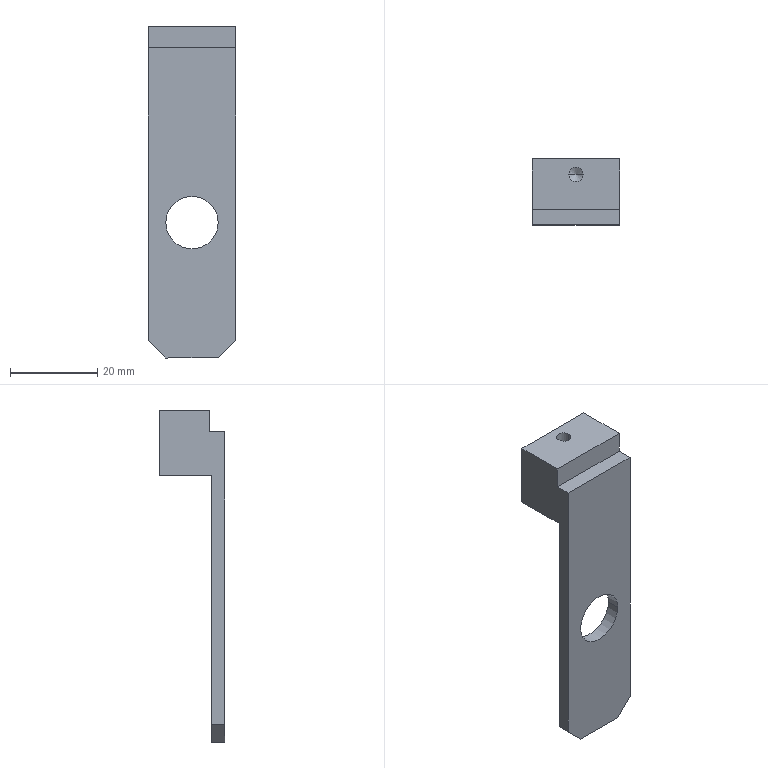Component | SolidWorks | GbgbMagnetBlockFeederF8-1 | 1 solid | 20 faces | box 20 x 15 x 76 mm | volume 7185 mm3 | plane 13 | cylinder 5 | cone 2 | commonest cylinder face diameters 12 x3 3.3 x2
build123d program:
from build123d import *

# Parameters (mm, degrees)
SKETCH1_W             = 71
SKETCH1_H             = 20
BOSS_EXTRUDE1_DEPTH   = 3
SKETCH2_W             = 10
SKETCH2_H             = 20
BOSS_EXTRUDE2_DEPTH   = 12
SKETCH3_R             = 6
CUT_EXTRUDE1_DEPTH    = 12
SKETCH6_W             = 19
SKETCH6_H             = 3
SKETCH6_H_2           = 5
BOSS_EXTRUDE3_DEPTH   = 3
SKETCH7_W             = 19
SKETCH7_H             = 5
SKETCH7_H_2           = 3
CUT_EXTRUDE2_DEPTH    = 10
SKETCH11_W            = 20
SKETCH11_H            = 15
BOSS_EXTRUDE4_DEPTH   = 5
SKETCH8_W             = 20
SKETCH8_H             = 3.5
CUT_EXTRUDE3_DEPTH    = 5
SKETCH9_R             = 6
CUT_EXTRUDE4_DEPTH    = 12
CHAMFER1_SIZE         = 4
M4_TAPPED_HOLE1_D     = 3.3
M4_TAPPED_HOLE1_DEPTH = 10.1
M4_TAPPED_HOLE1_TIP   = 0.9914


with BuildPart() as part:
    # Sketch1 → Boss-Extrude1 (new body)
    with BuildSketch(Plane(origin=(0, 0, 0), x_dir=(1, 0, 0), z_dir=(0, 1, 0))):
        Rectangle(SKETCH1_W, SKETCH1_H)
    extrude(amount=BOSS_EXTRUDE1_DEPTH)

    # Sketch2 → Boss-Extrude2 (add)
    with BuildSketch(Plane(origin=(0, 3, 0), x_dir=(1, 0, 0), z_dir=(0, 1, 0))):
        with Locations((-30.5, 0)):
            Rectangle(SKETCH2_W, SKETCH2_H)
    extrude(amount=BOSS_EXTRUDE2_DEPTH)

    # Sketch3 → Cut-Extrude1 (cut)
    with BuildSketch(Plane(origin=(0, 3, 0), x_dir=(1, 0, 0), z_dir=(0, 1, 0))):
        with Locations(Location((4.5, 0, 0), (0, 0, 270))):
            Circle(SKETCH3_R)
    extrude(amount=-CUT_EXTRUDE1_DEPTH, mode=Mode.SUBTRACT)

    # Sketch6 → Boss-Extrude3 (add)
    with BuildSketch(Plane.XZ):
        with Locations((0, 11.5)):
            Rectangle(SKETCH6_W, SKETCH6_H)
        with Locations((0, -12.5)):
            Rectangle(SKETCH6_W, SKETCH6_H_2)
    extrude(amount=-BOSS_EXTRUDE3_DEPTH)

    # Sketch7 → Cut-Extrude2 (cut)
    with BuildSketch(Plane(origin=(0, 3, 0), x_dir=(1, 0, 0), z_dir=(0, 1, 0))):
        with Locations((0, 12.5)):
            Rectangle(SKETCH7_W, SKETCH7_H)
        with Locations((0, -11.5)):
            Rectangle(SKETCH7_W, SKETCH7_H_2)
    extrude(amount=-CUT_EXTRUDE2_DEPTH, mode=Mode.SUBTRACT)

    # Sketch11 → Boss-Extrude4 (add)
    with BuildSketch(Plane.ZY.offset(35.5)):
        with Locations((0, 7.5)):
            Rectangle(SKETCH11_W, SKETCH11_H)
    extrude(amount=BOSS_EXTRUDE4_DEPTH)

    # Sketch8 → Cut-Extrude3 (cut)
    with BuildSketch(Plane.ZY.offset(40.5)):
        with Locations((0, 1.75)):
            Rectangle(SKETCH8_W, SKETCH8_H)
    extrude(amount=-CUT_EXTRUDE3_DEPTH, mode=Mode.SUBTRACT)

    # Sketch9 → Cut-Extrude4 (cut)
    with BuildSketch(Plane(origin=(0, 15, 0), x_dir=(1, 0, 0), z_dir=(0, 1, 0))):
        with Locations((-21.5, 0)):
            Circle(SKETCH9_R)
    extrude(amount=-CUT_EXTRUDE4_DEPTH, mode=Mode.SUBTRACT)

    # Chamfer1
    chamfer1_edges = [part.edges().sort_by_distance(p)[0] for p in [
        (35.5, 1.5, -10),
        (35.5, 1.5, 10),
    ]]
    chamfer(chamfer1_edges, length=CHAMFER1_SIZE)

    # M4 Tapped Hole1
    with Locations(Plane(origin=(-40.5, 4.795, -4.101), x_dir=(0, 0, 1), z_dir=(-1, 0, 0))):
        with Locations((4.101, 6.655)):
            Hole(M4_TAPPED_HOLE1_D / 2, depth=M4_TAPPED_HOLE1_DEPTH)
            with Locations((0, 0, -(M4_TAPPED_HOLE1_DEPTH + M4_TAPPED_HOLE1_TIP / 2))):  # 118° drill point
                Cone(0, M4_TAPPED_HOLE1_D / 2, M4_TAPPED_HOLE1_TIP, mode=Mode.SUBTRACT)


solid = part.part

# Placed as in the assembly
solid = solid.moved(Location((80.446, 384.34, 412.732), (0, 90, 0)))
STEP:
#1=COLOUR_RGB('',0.7922,0.8196,0.9333);
#2=FILL_AREA_STYLE_COLOUR('',#1);
#3=FILL_AREA_STYLE('',(#2));
#4=SURFACE_STYLE_FILL_AREA(#3);
#5=SURFACE_SIDE_STYLE('',(#4));
#6=SURFACE_STYLE_USAGE(.BOTH.,#5);
#7=PRESENTATION_STYLE_ASSIGNMENT((#6));
#8=CARTESIAN_POINT('',(3.102,15.582,17.446));
#9=VERTEX_POINT('',#8);
#10=CARTESIAN_POINT('',(3.232,15.582,17.446));
#11=VERTEX_POINT('',#10);
#12=CARTESIAN_POINT('',(3.167,15.582,17.446));
#13=DIRECTION('',(0.,0.,1.));
#14=DIRECTION('',(1.,0.,0.));
#15=AXIS2_PLACEMENT_3D('',#12,#13,#14);
#16=CIRCLE('',#15,0.06496);
#17=EDGE_CURVE('',#9,#11,#16,.T.);
#18=ORIENTED_EDGE('',*,*,#17,.F.);
#19=CARTESIAN_POINT('',(3.102,15.582,17.844));
#20=VERTEX_POINT('',#19);
#21=CARTESIAN_POINT('',(3.102,15.582,17.844));
#22=DIRECTION('',(0.,0.,1.));
#23=VECTOR('',#22,39.37);
#24=LINE('',#21,#23);
#25=EDGE_CURVE('',#9,#20,#24,.T.);
#26=ORIENTED_EDGE('',*,*,#25,.T.);
#27=CARTESIAN_POINT('',(3.232,15.582,17.844));
#28=VERTEX_POINT('',#27);
#29=CARTESIAN_POINT('',(3.167,15.582,17.844));
#30=DIRECTION('',(0.,0.,1.));
#31=DIRECTION('',(1.,0.,0.));
#32=AXIS2_PLACEMENT_3D('',#29,#30,#31);
#33=CIRCLE('',#32,0.06496);
#34=EDGE_CURVE('',#20,#28,#33,.T.);
#35=ORIENTED_EDGE('',*,*,#34,.T.);
#36=CARTESIAN_POINT('',(3.232,15.582,17.844));
#37=DIRECTION('',(0.,0.,1.));
#38=VECTOR('',#37,39.37);
#39=LINE('',#36,#38);
#40=EDGE_CURVE('',#11,#28,#39,.T.);
#41=ORIENTED_EDGE('',*,*,#40,.F.);
#42=EDGE_LOOP('',(#18,#26,#35,#41));
#43=FACE_OUTER_BOUND('',#42,.T.);
#44=CARTESIAN_POINT('',(3.167,15.582,17.844));
#45=DIRECTION('',(0.,0.,1.));
#46=DIRECTION('',(1.,0.,0.));
#47=AXIS2_PLACEMENT_3D('',#44,#45,#46);
#48=CYLINDRICAL_SURFACE('',#47,0.06496);
#49=ADVANCED_FACE('',(#43),#48,.F.);
#50=CARTESIAN_POINT('',(3.167,15.582,17.407));
#51=VERTEX_POINT('',#50);
#52=CARTESIAN_POINT('',(3.232,15.582,17.446));
#53=DIRECTION('',(0.8572,0.,0.515));
#54=VECTOR('',#53,39.37);
#55=LINE('',#52,#54);
#56=EDGE_CURVE('',#51,#11,#55,.T.);
#57=ORIENTED_EDGE('',*,*,#56,.F.);
#58=CARTESIAN_POINT('',(3.102,15.582,17.446));
#59=DIRECTION('',(-0.8572,-0.,0.515));
#60=VECTOR('',#59,39.37);
#61=LINE('',#58,#60);
#62=EDGE_CURVE('',#51,#9,#61,.T.);
#63=ORIENTED_EDGE('',*,*,#62,.T.);
#64=ORIENTED_EDGE('',*,*,#17,.T.);
#65=EDGE_LOOP('',(#57,#63,#64));
#66=FACE_OUTER_BOUND('',#65,.T.);
#67=CARTESIAN_POINT('',(3.167,15.582,17.446));
#68=DIRECTION('',(0.,0.,1.));
#69=DIRECTION('',(1.,0.,0.));
#70=AXIS2_PLACEMENT_3D('',#67,#68,#69);
#71=CONICAL_SURFACE('',#70,0.06496,1.03);
#72=ADVANCED_FACE('',(#66),#71,.F.);
#73=CARTESIAN_POINT('',(3.403,15.132,16.072));
#74=VERTEX_POINT('',#73);
#75=CARTESIAN_POINT('',(2.931,15.132,16.072));
#76=VERTEX_POINT('',#75);
#77=CARTESIAN_POINT('',(3.167,15.132,16.072));
#78=DIRECTION('',(0.,-1.,0.));
#79=DIRECTION('',(-1.,0.,0.));
#80=AXIS2_PLACEMENT_3D('',#77,#78,#79);
#81=CIRCLE('',#80,0.2362);
#82=EDGE_CURVE('',#74,#76,#81,.T.);
#83=ORIENTED_EDGE('',*,*,#82,.T.);
#84=CARTESIAN_POINT('',(2.931,15.25,16.072));
#85=VERTEX_POINT('',#84);
#86=CARTESIAN_POINT('',(2.931,14.777,16.072));
#87=DIRECTION('',(-0.,1.,-0.));
#88=VECTOR('',#87,39.37);
#89=LINE('',#86,#88);
#90=EDGE_CURVE('',#76,#85,#89,.T.);
#91=ORIENTED_EDGE('',*,*,#90,.T.);
#92=CARTESIAN_POINT('',(3.403,15.25,16.072));
#93=VERTEX_POINT('',#92);
#94=CARTESIAN_POINT('',(3.167,15.25,16.072));
#95=DIRECTION('',(-0.,1.,-0.));
#96=DIRECTION('',(1.,0.,0.));
#97=AXIS2_PLACEMENT_3D('',#94,#95,#96);
#98=CIRCLE('',#97,0.2362);
#99=EDGE_CURVE('',#85,#93,#98,.T.);
#100=ORIENTED_EDGE('',*,*,#99,.T.);
#101=CARTESIAN_POINT('',(3.403,14.777,16.072));
#102=DIRECTION('',(-0.,1.,-0.));
#103=VECTOR('',#102,39.37);
#104=LINE('',#101,#103);
#105=EDGE_CURVE('',#74,#93,#104,.T.);
#106=ORIENTED_EDGE('',*,*,#105,.F.);
#107=EDGE_LOOP('',(#83,#91,#100,#106));
#108=FACE_OUTER_BOUND('',#107,.T.);
#109=CARTESIAN_POINT('',(3.167,14.777,16.072));
#110=DIRECTION('',(-0.,1.,-0.));
#111=DIRECTION('',(1.,0.,0.));
#112=AXIS2_PLACEMENT_3D('',#109,#110,#111);
#113=CYLINDRICAL_SURFACE('',#112,0.2362);
#114=ADVANCED_FACE('',(#108),#113,.F.);
#115=CARTESIAN_POINT('',(3.561,15.25,17.253));
#116=VERTEX_POINT('',#115);
#117=CARTESIAN_POINT('',(3.343,15.25,17.253));
#118=VERTEX_POINT('',#117);
#119=CARTESIAN_POINT('',(2.773,15.25,17.253));
#120=DIRECTION('',(-1.,-0.,0.));
#121=VECTOR('',#120,39.37);
#122=LINE('',#119,#121);
#123=EDGE_CURVE('',#116,#118,#122,.T.);
#124=ORIENTED_EDGE('',*,*,#123,.T.);
#125=CARTESIAN_POINT('',(3.343,15.722,17.253));
#126=VERTEX_POINT('',#125);
#127=CARTESIAN_POINT('',(3.343,14.581,17.253));
#128=DIRECTION('',(-0.,1.,-0.));
#129=VECTOR('',#128,39.37);
#130=LINE('',#127,#129);
#131=EDGE_CURVE('',#118,#126,#130,.T.);
#132=ORIENTED_EDGE('',*,*,#131,.T.);
#133=CARTESIAN_POINT('',(3.561,15.722,17.253));
#134=VERTEX_POINT('',#133);
#135=CARTESIAN_POINT('',(2.773,15.722,17.253));
#136=DIRECTION('',(-1.,-0.,0.));
#137=VECTOR('',#136,39.37);
#138=LINE('',#135,#137);
#139=EDGE_CURVE('',#134,#126,#138,.T.);
#140=ORIENTED_EDGE('',*,*,#139,.F.);
#141=CARTESIAN_POINT('',(3.561,15.722,17.253));
#142=DIRECTION('',(0.,-1.,0.));
#143=VECTOR('',#142,39.37);
#144=LINE('',#141,#143);
#145=EDGE_CURVE('',#134,#116,#144,.T.);
#146=ORIENTED_EDGE('',*,*,#145,.T.);
#147=EDGE_LOOP('',(#124,#132,#140,#146));
#148=FACE_OUTER_BOUND('',#147,.T.);
#149=CARTESIAN_POINT('',(2.773,15.722,17.253));
#150=DIRECTION('',(0.,0.,1.));
#151=DIRECTION('',(1.,0.,-0.));
#152=AXIS2_PLACEMENT_3D('',#149,#150,#151);
#153=PLANE('',#152);
#154=ADVANCED_FACE('',(#148),#153,.F.);
#155=CARTESIAN_POINT('',(3.167,15.25,16.072));
#156=DIRECTION('',(-0.,1.,-0.));
#157=DIRECTION('',(1.,0.,0.));
#158=AXIS2_PLACEMENT_3D('',#155,#156,#157);
#159=CIRCLE('',#158,0.2362);
#160=EDGE_CURVE('',#93,#85,#159,.T.);
#161=ORIENTED_EDGE('',*,*,#160,.F.);
#162=ORIENTED_EDGE('',*,*,#99,.F.);
#163=EDGE_LOOP('',(#161,#162));
#164=FACE_BOUND('',#163,.T.);
#165=CARTESIAN_POINT('',(3.403,15.25,14.852));
#166=VERTEX_POINT('',#165);
#167=CARTESIAN_POINT('',(2.931,15.25,14.852));
#168=VERTEX_POINT('',#167);
#169=CARTESIAN_POINT('',(2.773,15.25,14.852));
#170=DIRECTION('',(-1.,-0.,-0.));
#171=VECTOR('',#170,39.37);
#172=LINE('',#169,#171);
#173=EDGE_CURVE('',#166,#168,#172,.T.);
#174=ORIENTED_EDGE('',*,*,#173,.T.);
#175=CARTESIAN_POINT('',(2.773,15.25,15.009));
#176=VERTEX_POINT('',#175);
#177=CARTESIAN_POINT('',(2.773,15.25,15.009));
#178=DIRECTION('',(-0.7071,-0.,0.7071));
#179=VECTOR('',#178,39.37);
#180=LINE('',#177,#179);
#181=EDGE_CURVE('',#168,#176,#180,.T.);
#182=ORIENTED_EDGE('',*,*,#181,.T.);
#183=CARTESIAN_POINT('',(2.773,15.25,17.253));
#184=VERTEX_POINT('',#183);
#185=CARTESIAN_POINT('',(2.773,15.25,14.852));
#186=DIRECTION('',(0.,0.,1.));
#187=VECTOR('',#186,39.37);
#188=LINE('',#185,#187);
#189=EDGE_CURVE('',#176,#184,#188,.T.);
#190=ORIENTED_EDGE('',*,*,#189,.T.);
#191=CARTESIAN_POINT('',(2.991,15.25,17.253));
#192=VERTEX_POINT('',#191);
#193=CARTESIAN_POINT('',(2.773,15.25,17.253));
#194=DIRECTION('',(-1.,-0.,0.));
#195=VECTOR('',#194,39.37);
#196=LINE('',#193,#195);
#197=EDGE_CURVE('',#192,#184,#196,.T.);
#198=ORIENTED_EDGE('',*,*,#197,.F.);
#199=CARTESIAN_POINT('',(3.167,15.25,17.096));
#200=DIRECTION('',(-0.,1.,-0.));
#201=DIRECTION('',(-1.,0.,0.));
#202=AXIS2_PLACEMENT_3D('',#199,#200,#201);
#203=CIRCLE('',#202,0.2362);
#204=EDGE_CURVE('',#192,#118,#203,.T.);
#205=ORIENTED_EDGE('',*,*,#204,.T.);
#206=ORIENTED_EDGE('',*,*,#123,.F.);
#207=CARTESIAN_POINT('',(3.561,15.25,15.009));
#208=VERTEX_POINT('',#207);
#209=CARTESIAN_POINT('',(3.561,15.25,14.852));
#210=DIRECTION('',(-0.,-0.,-1.));
#211=VECTOR('',#210,39.37);
#212=LINE('',#209,#211);
#213=EDGE_CURVE('',#116,#208,#212,.T.);
#214=ORIENTED_EDGE('',*,*,#213,.T.);
#215=CARTESIAN_POINT('',(3.403,15.25,14.852));
#216=DIRECTION('',(-0.7071,-0.,-0.7071));
#217=VECTOR('',#216,39.37);
#218=LINE('',#215,#217);
#219=EDGE_CURVE('',#208,#166,#218,.T.);
#220=ORIENTED_EDGE('',*,*,#219,.T.);
#221=EDGE_LOOP('',(#174,#182,#190,#198,#205,#206,#214,#220));
#222=FACE_OUTER_BOUND('',#221,.T.);
#223=CARTESIAN_POINT('',(3.167,15.25,16.249));
#224=DIRECTION('',(0.,-1.,0.));
#225=DIRECTION('',(-1.,-0.,0.));
#226=AXIS2_PLACEMENT_3D('',#223,#224,#225);
#227=PLANE('',#226);
#228=ADVANCED_FACE('',(#164,#222),#227,.F.);
#229=CARTESIAN_POINT('',(3.561,15.132,17.647));
#230=VERTEX_POINT('',#229);
#231=CARTESIAN_POINT('',(3.561,15.132,15.009));
#232=VERTEX_POINT('',#231);
#233=CARTESIAN_POINT('',(3.561,15.132,14.852));
#234=DIRECTION('',(-0.,-0.,-1.));
#235=VECTOR('',#234,39.37);
#236=LINE('',#233,#235);
#237=EDGE_CURVE('',#230,#232,#236,.T.);
#238=ORIENTED_EDGE('',*,*,#237,.T.);
#239=CARTESIAN_POINT('',(3.561,15.25,15.009));
#240=DIRECTION('',(-0.,1.,-0.));
#241=VECTOR('',#240,39.37);
#242=LINE('',#239,#241);
#243=EDGE_CURVE('',#232,#208,#242,.T.);
#244=ORIENTED_EDGE('',*,*,#243,.T.);
#245=ORIENTED_EDGE('',*,*,#213,.F.);
#246=ORIENTED_EDGE('',*,*,#145,.F.);
#247=CARTESIAN_POINT('',(3.561,15.722,17.844));
#248=VERTEX_POINT('',#247);
#249=CARTESIAN_POINT('',(3.561,15.722,17.647));
#250=DIRECTION('',(-0.,-0.,-1.));
#251=VECTOR('',#250,39.37);
#252=LINE('',#249,#251);
#253=EDGE_CURVE('',#248,#134,#252,.T.);
#254=ORIENTED_EDGE('',*,*,#253,.F.);
#255=CARTESIAN_POINT('',(3.561,15.269,17.844));
#256=VERTEX_POINT('',#255);
#257=CARTESIAN_POINT('',(3.561,15.722,17.844));
#258=DIRECTION('',(-0.,1.,-0.));
#259=VECTOR('',#258,39.37);
#260=LINE('',#257,#259);
#261=EDGE_CURVE('',#256,#248,#260,.T.);
#262=ORIENTED_EDGE('',*,*,#261,.F.);
#263=CARTESIAN_POINT('',(3.561,15.269,17.647));
#264=VERTEX_POINT('',#263);
#265=CARTESIAN_POINT('',(3.561,15.269,17.647));
#266=DIRECTION('',(0.,0.,1.));
#267=VECTOR('',#266,39.37);
#268=LINE('',#265,#267);
#269=EDGE_CURVE('',#264,#256,#268,.T.);
#270=ORIENTED_EDGE('',*,*,#269,.F.);
#271=CARTESIAN_POINT('',(3.561,15.132,17.647));
#272=DIRECTION('',(-0.,1.,-0.));
#273=VECTOR('',#272,39.37);
#274=LINE('',#271,#273);
#275=EDGE_CURVE('',#230,#264,#274,.T.);
#276=ORIENTED_EDGE('',*,*,#275,.F.);
#277=EDGE_LOOP('',(#238,#244,#245,#246,#254,#262,#270,#276));
#278=FACE_OUTER_BOUND('',#277,.T.);
#279=CARTESIAN_POINT('',(3.561,15.25,14.852));
#280=DIRECTION('',(-1.,-0.,0.));
#281=DIRECTION('',(0.,0.,1.));
#282=AXIS2_PLACEMENT_3D('',#279,#280,#281);
#283=PLANE('',#282);
#284=ADVANCED_FACE('',(#278),#283,.F.);
#285=CARTESIAN_POINT('',(3.403,15.132,14.852));
#286=VERTEX_POINT('',#285);
#287=CARTESIAN_POINT('',(2.931,15.132,14.852));
#288=VERTEX_POINT('',#287);
#289=CARTESIAN_POINT('',(2.773,15.132,14.852));
#290=DIRECTION('',(-1.,-0.,-0.));
#291=VECTOR('',#290,39.37);
#292=LINE('',#289,#291);
#293=EDGE_CURVE('',#286,#288,#292,.T.);
#294=ORIENTED_EDGE('',*,*,#293,.T.);
#295=CARTESIAN_POINT('',(2.931,15.25,14.852));
#296=DIRECTION('',(-0.,1.,-0.));
#297=VECTOR('',#296,39.37);
#298=LINE('',#295,#297);
#299=EDGE_CURVE('',#288,#168,#298,.T.);
#300=ORIENTED_EDGE('',*,*,#299,.T.);
#301=ORIENTED_EDGE('',*,*,#173,.F.);
#302=CARTESIAN_POINT('',(3.403,15.25,14.852));
#303=DIRECTION('',(0.,-1.,0.));
#304=VECTOR('',#303,39.37);
#305=LINE('',#302,#304);
#306=EDGE_CURVE('',#166,#286,#305,.T.);
#307=ORIENTED_EDGE('',*,*,#306,.T.);
#308=EDGE_LOOP('',(#294,#300,#301,#307));
#309=FACE_OUTER_BOUND('',#308,.T.);
#310=CARTESIAN_POINT('',(2.773,15.25,14.852));
#311=DIRECTION('',(-0.,-0.,1.));
#312=DIRECTION('',(1.,0.,0.));
#313=AXIS2_PLACEMENT_3D('',#310,#311,#312);
#314=PLANE('',#313);
#315=ADVANCED_FACE('',(#309),#314,.F.);
#316=ORIENTED_EDGE('',*,*,#189,.F.);
#317=CARTESIAN_POINT('',(2.773,15.132,15.009));
#318=VERTEX_POINT('',#317);
#319=CARTESIAN_POINT('',(2.773,15.25,15.009));
#320=DIRECTION('',(0.,-1.,0.));
#321=VECTOR('',#320,39.37);
#322=LINE('',#319,#321);
#323=EDGE_CURVE('',#176,#318,#322,.T.);
#324=ORIENTED_EDGE('',*,*,#323,.T.);
#325=CARTESIAN_POINT('',(2.773,15.132,17.647));
#326=VERTEX_POINT('',#325);
#327=CARTESIAN_POINT('',(2.773,15.132,14.852));
#328=DIRECTION('',(0.,0.,1.));
#329=VECTOR('',#328,39.37);
#330=LINE('',#327,#329);
#331=EDGE_CURVE('',#318,#326,#330,.T.);
#332=ORIENTED_EDGE('',*,*,#331,.T.);
#333=CARTESIAN_POINT('',(2.773,15.269,17.647));
#334=VERTEX_POINT('',#333);
#335=CARTESIAN_POINT('',(2.773,15.132,17.647));
#336=DIRECTION('',(0.,-1.,0.));
#337=VECTOR('',#336,39.37);
#338=LINE('',#335,#337);
#339=EDGE_CURVE('',#334,#326,#338,.T.);
#340=ORIENTED_EDGE('',*,*,#339,.F.);
#341=CARTESIAN_POINT('',(2.773,15.269,17.844));
#342=VERTEX_POINT('',#341);
#343=CARTESIAN_POINT('',(2.773,15.269,17.647));
#344=DIRECTION('',(0.,0.,1.));
#345=VECTOR('',#344,39.37);
#346=LINE('',#343,#345);
#347=EDGE_CURVE('',#334,#342,#346,.T.);
#348=ORIENTED_EDGE('',*,*,#347,.T.);
#349=CARTESIAN_POINT('',(2.773,15.722,17.844));
#350=VERTEX_POINT('',#349);
#351=CARTESIAN_POINT('',(2.773,15.722,17.844));
#352=DIRECTION('',(0.,-1.,0.));
#353=VECTOR('',#352,39.37);
#354=LINE('',#351,#353);
#355=EDGE_CURVE('',#350,#342,#354,.T.);
#356=ORIENTED_EDGE('',*,*,#355,.F.);
#357=CARTESIAN_POINT('',(2.773,15.722,17.253));
#358=VERTEX_POINT('',#357);
#359=CARTESIAN_POINT('',(2.773,15.722,17.647));
#360=DIRECTION('',(0.,0.,1.));
#361=VECTOR('',#360,39.37);
#362=LINE('',#359,#361);
#363=EDGE_CURVE('',#358,#350,#362,.T.);
#364=ORIENTED_EDGE('',*,*,#363,.F.);
#365=CARTESIAN_POINT('',(2.773,15.722,17.253));
#366=DIRECTION('',(0.,-1.,0.));
#367=VECTOR('',#366,39.37);
#368=LINE('',#365,#367);
#369=EDGE_CURVE('',#358,#184,#368,.T.);
#370=ORIENTED_EDGE('',*,*,#369,.T.);
#371=EDGE_LOOP('',(#316,#324,#332,#340,#348,#356,#364,#370));
#372=FACE_OUTER_BOUND('',#371,.T.);
#373=CARTESIAN_POINT('',(2.773,15.25,14.852));
#374=DIRECTION('',(1.,0.,-0.));
#375=DIRECTION('',(-0.,-0.,-1.));
#376=AXIS2_PLACEMENT_3D('',#373,#374,#375);
#377=PLANE('',#376);
#378=ADVANCED_FACE('',(#372),#377,.F.);
#379=ORIENTED_EDGE('',*,*,#331,.F.);
#380=CARTESIAN_POINT('',(2.35,15.132,15.432));
#381=DIRECTION('',(0.7071,0.,-0.7071));
#382=VECTOR('',#381,39.37);
#383=LINE('',#380,#382);
#384=EDGE_CURVE('',#318,#288,#383,.T.);
#385=ORIENTED_EDGE('',*,*,#384,.T.);
#386=ORIENTED_EDGE('',*,*,#293,.F.);
#387=CARTESIAN_POINT('',(3.984,15.132,15.432));
#388=DIRECTION('',(0.7071,0.,0.7071));
#389=VECTOR('',#388,39.37);
#390=LINE('',#387,#389);
#391=EDGE_CURVE('',#286,#232,#390,.T.);
#392=ORIENTED_EDGE('',*,*,#391,.T.);
#393=ORIENTED_EDGE('',*,*,#237,.F.);
#394=CARTESIAN_POINT('',(2.773,15.132,17.647));
#395=DIRECTION('',(1.,0.,-0.));
#396=VECTOR('',#395,39.37);
#397=LINE('',#394,#396);
#398=EDGE_CURVE('',#326,#230,#397,.T.);
#399=ORIENTED_EDGE('',*,*,#398,.F.);
#400=EDGE_LOOP('',(#379,#385,#386,#392,#393,#399));
#401=FACE_OUTER_BOUND('',#400,.T.);
#402=ORIENTED_EDGE('',*,*,#82,.F.);
#403=CARTESIAN_POINT('',(3.167,15.132,16.072));
#404=DIRECTION('',(0.,-1.,0.));
#405=DIRECTION('',(-1.,0.,0.));
#406=AXIS2_PLACEMENT_3D('',#403,#404,#405);
#407=CIRCLE('',#406,0.2362);
#408=EDGE_CURVE('',#76,#74,#407,.T.);
#409=ORIENTED_EDGE('',*,*,#408,.F.);
#410=EDGE_LOOP('',(#402,#409));
#411=FACE_BOUND('',#410,.T.);
#412=CARTESIAN_POINT('',(3.167,15.132,16.249));
#413=DIRECTION('',(0.,-1.,0.));
#414=DIRECTION('',(-1.,-0.,0.));
#415=AXIS2_PLACEMENT_3D('',#412,#413,#414);
#416=PLANE('',#415);
#417=ADVANCED_FACE('',(#401,#411),#416,.T.);
#418=CARTESIAN_POINT('',(2.991,15.722,17.253));
#419=VERTEX_POINT('',#418);
#420=CARTESIAN_POINT('',(2.773,15.722,17.253));
#421=DIRECTION('',(-1.,-0.,0.));
#422=VECTOR('',#421,39.37);
#423=LINE('',#420,#422);
#424=EDGE_CURVE('',#419,#358,#423,.T.);
#425=ORIENTED_EDGE('',*,*,#424,.F.);
#426=CARTESIAN_POINT('',(2.991,14.581,17.253));
#427=DIRECTION('',(0.,-1.,0.));
#428=VECTOR('',#427,39.37);
#429=LINE('',#426,#428);
#430=EDGE_CURVE('',#419,#192,#429,.T.);
#431=ORIENTED_EDGE('',*,*,#430,.T.);
#432=ORIENTED_EDGE('',*,*,#197,.T.);
#433=ORIENTED_EDGE('',*,*,#369,.F.);
#434=EDGE_LOOP('',(#425,#431,#432,#433));
#435=FACE_OUTER_BOUND('',#434,.T.);
#436=CARTESIAN_POINT('',(2.773,15.722,17.253));
#437=DIRECTION('',(0.,0.,1.));
#438=DIRECTION('',(1.,0.,-0.));
#439=AXIS2_PLACEMENT_3D('',#436,#437,#438);
#440=PLANE('',#439);
#441=ADVANCED_FACE('',(#435),#440,.F.);
#442=CARTESIAN_POINT('',(3.167,15.722,17.096));
#443=DIRECTION('',(-0.,1.,-0.));
#444=DIRECTION('',(1.,0.,0.));
#445=AXIS2_PLACEMENT_3D('',#442,#443,#444);
#446=CIRCLE('',#445,0.2362);
#447=EDGE_CURVE('',#419,#126,#446,.T.);
#448=ORIENTED_EDGE('',*,*,#447,.F.);
#449=ORIENTED_EDGE('',*,*,#424,.T.);
#450=ORIENTED_EDGE('',*,*,#363,.T.);
#451=CARTESIAN_POINT('',(2.773,15.722,17.844));
#452=DIRECTION('',(-1.,-0.,0.));
#453=VECTOR('',#452,39.37);
#454=LINE('',#451,#453);
#455=EDGE_CURVE('',#248,#350,#454,.T.);
#456=ORIENTED_EDGE('',*,*,#455,.F.);
#457=ORIENTED_EDGE('',*,*,#253,.T.);
#458=ORIENTED_EDGE('',*,*,#139,.T.);
#459=EDGE_LOOP('',(#448,#449,#450,#456,#457,#458));
#460=FACE_OUTER_BOUND('',#459,.T.);
#461=CARTESIAN_POINT('',(3.167,15.722,16.249));
#462=DIRECTION('',(-0.,1.,-0.));
#463=DIRECTION('',(1.,0.,-0.));
#464=AXIS2_PLACEMENT_3D('',#461,#462,#463);
#465=PLANE('',#464);
#466=ADVANCED_FACE('',(#460),#465,.T.);
#467=ORIENTED_EDGE('',*,*,#90,.F.);
#468=ORIENTED_EDGE('',*,*,#408,.T.);
#469=ORIENTED_EDGE('',*,*,#105,.T.);
#470=ORIENTED_EDGE('',*,*,#160,.T.);
#471=EDGE_LOOP('',(#467,#468,#469,#470));
#472=FACE_OUTER_BOUND('',#471,.T.);
#473=CARTESIAN_POINT('',(3.167,14.777,16.072));
#474=DIRECTION('',(-0.,1.,-0.));
#475=DIRECTION('',(1.,0.,0.));
#476=AXIS2_PLACEMENT_3D('',#473,#474,#475);
#477=CYLINDRICAL_SURFACE('',#476,0.2362);
#478=ADVANCED_FACE('',(#472),#477,.F.);
#479=CARTESIAN_POINT('',(3.167,15.582,17.844));
#480=DIRECTION('',(0.,0.,1.));
#481=DIRECTION('',(1.,0.,0.));
#482=AXIS2_PLACEMENT_3D('',#479,#480,#481);
#483=CIRCLE('',#482,0.06496);
#484=EDGE_CURVE('',#28,#20,#483,.T.);
#485=ORIENTED_EDGE('',*,*,#484,.F.);
#486=ORIENTED_EDGE('',*,*,#34,.F.);
#487=EDGE_LOOP('',(#485,#486));
#488=FACE_BOUND('',#487,.T.);
#489=CARTESIAN_POINT('',(2.773,15.269,17.844));
#490=DIRECTION('',(-1.,-0.,0.));
#491=VECTOR('',#490,39.37);
#492=LINE('',#489,#491);
#493=EDGE_CURVE('',#256,#342,#492,.T.);
#494=ORIENTED_EDGE('',*,*,#493,.F.);
#495=ORIENTED_EDGE('',*,*,#261,.T.);
#496=ORIENTED_EDGE('',*,*,#455,.T.);
#497=ORIENTED_EDGE('',*,*,#355,.T.);
#498=EDGE_LOOP('',(#494,#495,#496,#497));
#499=FACE_OUTER_BOUND('',#498,.T.);
#500=CARTESIAN_POINT('',(3.167,15.132,17.844));
#501=DIRECTION('',(0.,0.,1.));
#502=DIRECTION('',(1.,0.,-0.));
#503=AXIS2_PLACEMENT_3D('',#500,#501,#502);
#504=PLANE('',#503);
#505=ADVANCED_FACE('',(#488,#499),#504,.T.);
#506=ORIENTED_EDGE('',*,*,#493,.T.);
#507=ORIENTED_EDGE('',*,*,#347,.F.);
#508=CARTESIAN_POINT('',(2.773,15.269,17.647));
#509=DIRECTION('',(-1.,-0.,0.));
#510=VECTOR('',#509,39.37);
#511=LINE('',#508,#510);
#512=EDGE_CURVE('',#264,#334,#511,.T.);
#513=ORIENTED_EDGE('',*,*,#512,.F.);
#514=ORIENTED_EDGE('',*,*,#269,.T.);
#515=EDGE_LOOP('',(#506,#507,#513,#514));
#516=FACE_OUTER_BOUND('',#515,.T.);
#517=CARTESIAN_POINT('',(2.773,15.269,17.647));
#518=DIRECTION('',(-0.,1.,-0.));
#519=DIRECTION('',(1.,0.,-0.));
#520=AXIS2_PLACEMENT_3D('',#517,#518,#519);
#521=PLANE('',#520);
#522=ADVANCED_FACE('',(#516),#521,.F.);
#523=ORIENTED_EDGE('',*,*,#339,.T.);
#524=ORIENTED_EDGE('',*,*,#398,.T.);
#525=ORIENTED_EDGE('',*,*,#275,.T.);
#526=ORIENTED_EDGE('',*,*,#512,.T.);
#527=EDGE_LOOP('',(#523,#524,#525,#526));
#528=FACE_OUTER_BOUND('',#527,.T.);
#529=CARTESIAN_POINT('',(3.167,15.132,17.647));
#530=DIRECTION('',(-0.,-0.,-1.));
#531=DIRECTION('',(-1.,-0.,0.));
#532=AXIS2_PLACEMENT_3D('',#529,#530,#531);
#533=PLANE('',#532);
#534=ADVANCED_FACE('',(#528),#533,.F.);
#535=ORIENTED_EDGE('',*,*,#204,.F.);
#536=ORIENTED_EDGE('',*,*,#430,.F.);
#537=ORIENTED_EDGE('',*,*,#447,.T.);
#538=ORIENTED_EDGE('',*,*,#131,.F.);
#539=EDGE_LOOP('',(#535,#536,#537,#538));
#540=FACE_OUTER_BOUND('',#539,.T.);
#541=CARTESIAN_POINT('',(3.167,14.581,17.096));
#542=DIRECTION('',(-0.,1.,-0.));
#543=DIRECTION('',(1.,0.,0.));
#544=AXIS2_PLACEMENT_3D('',#541,#542,#543);
#545=CYLINDRICAL_SURFACE('',#544,0.2362);
#546=ADVANCED_FACE('',(#540),#545,.F.);
#547=ORIENTED_EDGE('',*,*,#181,.F.);
#548=ORIENTED_EDGE('',*,*,#299,.F.);
#549=ORIENTED_EDGE('',*,*,#384,.F.);
#550=ORIENTED_EDGE('',*,*,#323,.F.);
#551=EDGE_LOOP('',(#547,#548,#549,#550));
#552=FACE_OUTER_BOUND('',#551,.T.);
#553=CARTESIAN_POINT('',(2.773,15.25,15.009));
#554=DIRECTION('',(0.7071,0.,0.7071));
#555=DIRECTION('',(0.,-1.,0.));
#556=AXIS2_PLACEMENT_3D('',#553,#554,#555);
#557=PLANE('',#556);
#558=ADVANCED_FACE('',(#552),#557,.F.);
#559=ORIENTED_EDGE('',*,*,#219,.F.);
#560=ORIENTED_EDGE('',*,*,#243,.F.);
#561=ORIENTED_EDGE('',*,*,#391,.F.);
#562=ORIENTED_EDGE('',*,*,#306,.F.);
#563=EDGE_LOOP('',(#559,#560,#561,#562));
#564=FACE_OUTER_BOUND('',#563,.T.);
#565=CARTESIAN_POINT('',(3.403,15.25,14.852));
#566=DIRECTION('',(-0.7071,-0.,0.7071));
#567=DIRECTION('',(0.,-1.,0.));
#568=AXIS2_PLACEMENT_3D('',#565,#566,#567);
#569=PLANE('',#568);
#570=ADVANCED_FACE('',(#564),#569,.F.);
#571=ORIENTED_EDGE('',*,*,#62,.F.);
#572=ORIENTED_EDGE('',*,*,#56,.T.);
#573=CARTESIAN_POINT('',(3.167,15.582,17.446));
#574=DIRECTION('',(0.,0.,1.));
#575=DIRECTION('',(1.,0.,0.));
#576=AXIS2_PLACEMENT_3D('',#573,#574,#575);
#577=CIRCLE('',#576,0.06496);
#578=EDGE_CURVE('',#11,#9,#577,.T.);
#579=ORIENTED_EDGE('',*,*,#578,.T.);
#580=EDGE_LOOP('',(#571,#572,#579));
#581=FACE_OUTER_BOUND('',#580,.T.);
#582=CARTESIAN_POINT('',(3.167,15.582,17.446));
#583=DIRECTION('',(0.,0.,1.));
#584=DIRECTION('',(1.,0.,0.));
#585=AXIS2_PLACEMENT_3D('',#582,#583,#584);
#586=CONICAL_SURFACE('',#585,0.06496,1.03);
#587=ADVANCED_FACE('',(#581),#586,.F.);
#588=ORIENTED_EDGE('',*,*,#25,.F.);
#589=ORIENTED_EDGE('',*,*,#578,.F.);
#590=ORIENTED_EDGE('',*,*,#40,.T.);
#591=ORIENTED_EDGE('',*,*,#484,.T.);
#592=EDGE_LOOP('',(#588,#589,#590,#591));
#593=FACE_OUTER_BOUND('',#592,.T.);
#594=CARTESIAN_POINT('',(3.167,15.582,17.844));
#595=DIRECTION('',(0.,0.,1.));
#596=DIRECTION('',(1.,0.,0.));
#597=AXIS2_PLACEMENT_3D('',#594,#595,#596);
#598=CYLINDRICAL_SURFACE('',#597,0.06496);
#599=ADVANCED_FACE('',(#593),#598,.F.);
#600=CLOSED_SHELL('',(#49,#72,#114,#154,#228,#284,#315,#378,#417,#441,#466,#478,#505,#522,#534,#546,#558,#570,#587,#599));
#601=MANIFOLD_SOLID_BREP('',#600);
#602=STYLED_ITEM('',(#7),#601);
#603=PRESENTATION_LAYER_ASSIGNMENT('','',(#602));
#604=CARTESIAN_POINT('',(0.,0.,0.));
#605=DIRECTION('',(0.,0.,1.));
#606=DIRECTION('',(1.,0.,0.));
#607=AXIS2_PLACEMENT_3D('',#604,#605,#606);
#608=(LENGTH_UNIT()NAMED_UNIT(*)SI_UNIT($,.METRE.));
#609=LENGTH_MEASURE_WITH_UNIT(LENGTH_MEASURE(0.0254),#608);
#610=DIMENSIONAL_EXPONENTS(1.,0.,0.,0.,0.,0.,0.);
#611=(CONVERSION_BASED_UNIT('',#609)LENGTH_UNIT()NAMED_UNIT(#610));
#612=UNCERTAINTY_MEASURE_WITH_UNIT(LENGTH_MEASURE(0.00001),#611,'','');
#613=(NAMED_UNIT(*)PLANE_ANGLE_UNIT()SI_UNIT($,.RADIAN.));
#614=(NAMED_UNIT(*)SI_UNIT($,.STERADIAN.)SOLID_ANGLE_UNIT());
#615=(GEOMETRIC_REPRESENTATION_CONTEXT(3)GLOBAL_UNCERTAINTY_ASSIGNED_CONTEXT((#612))GLOBAL_UNIT_ASSIGNED_CONTEXT((#611,#613,#614))REPRESENTATION_CONTEXT('',''));
#616=ADVANCED_BREP_SHAPE_REPRESENTATION('',(#601,#607),#615);
#617=(LENGTH_UNIT()NAMED_UNIT(*)SI_UNIT($,.METRE.));
#618=LENGTH_MEASURE_WITH_UNIT(LENGTH_MEASURE(0.0254),#617);
#619=DIMENSIONAL_EXPONENTS(1.,0.,0.,0.,0.,0.,0.);
#620=(CONVERSION_BASED_UNIT('',#618)LENGTH_UNIT()NAMED_UNIT(#619));
#621=UNCERTAINTY_MEASURE_WITH_UNIT(LENGTH_MEASURE(0.00001),#620,'','');
#622=(NAMED_UNIT(*)PLANE_ANGLE_UNIT()SI_UNIT($,.RADIAN.));
#623=(NAMED_UNIT(*)SI_UNIT($,.STERADIAN.)SOLID_ANGLE_UNIT());
#624=(GEOMETRIC_REPRESENTATION_CONTEXT(3)GLOBAL_UNCERTAINTY_ASSIGNED_CONTEXT((#621))GLOBAL_UNIT_ASSIGNED_CONTEXT((#620,#622,#623))REPRESENTATION_CONTEXT('',''));
#625=MECHANICAL_DESIGN_GEOMETRIC_PRESENTATION_REPRESENTATION('',(#602),#624);